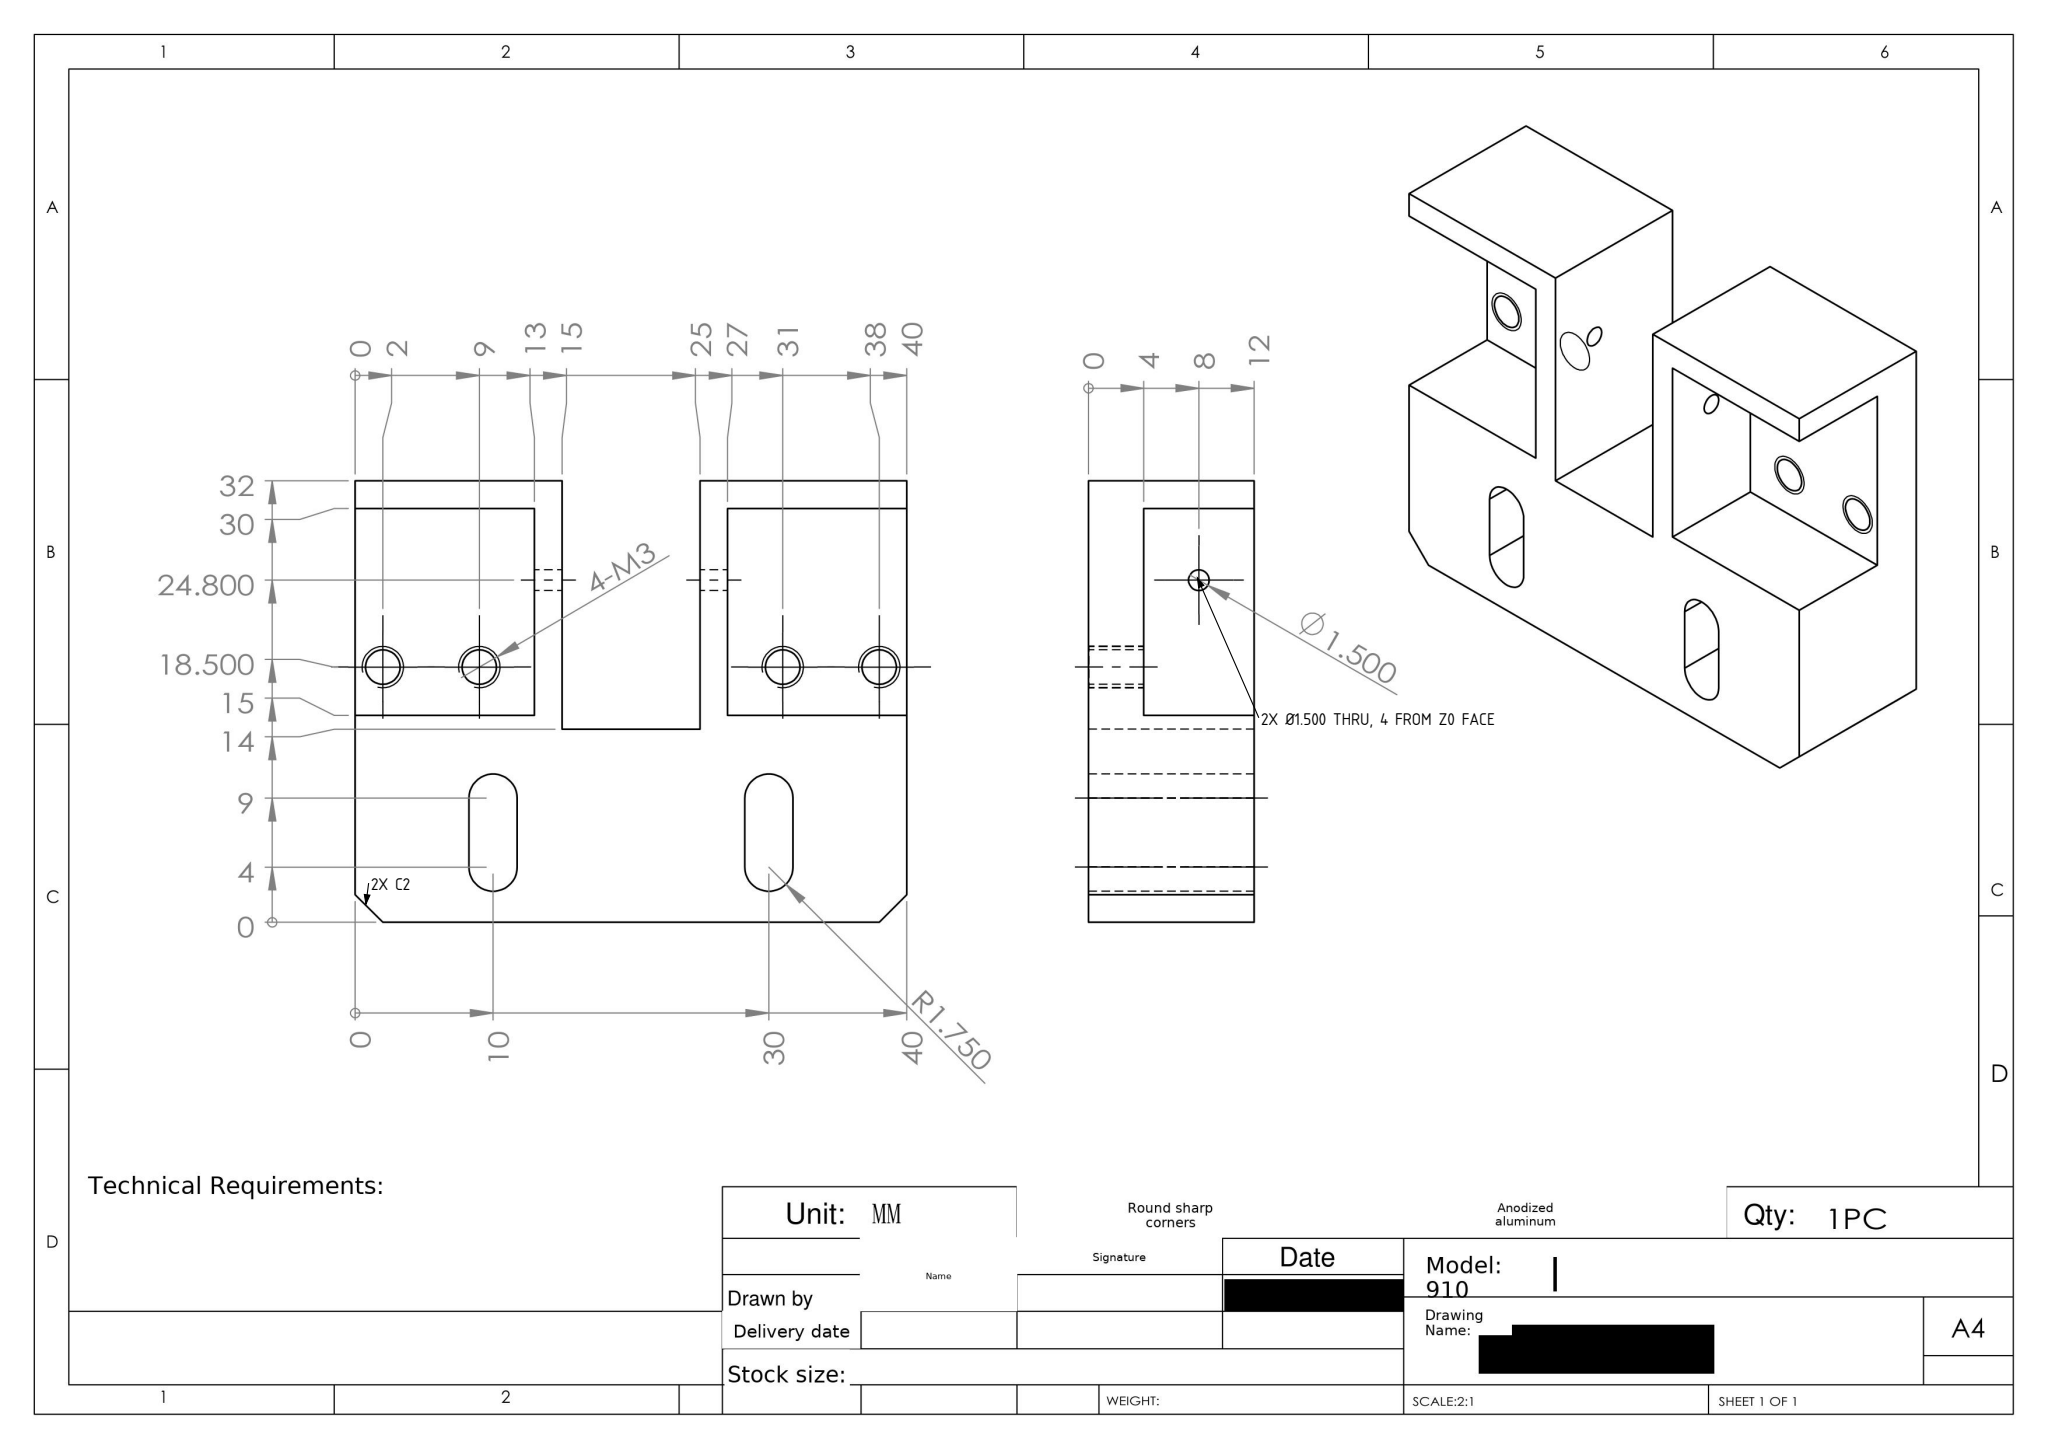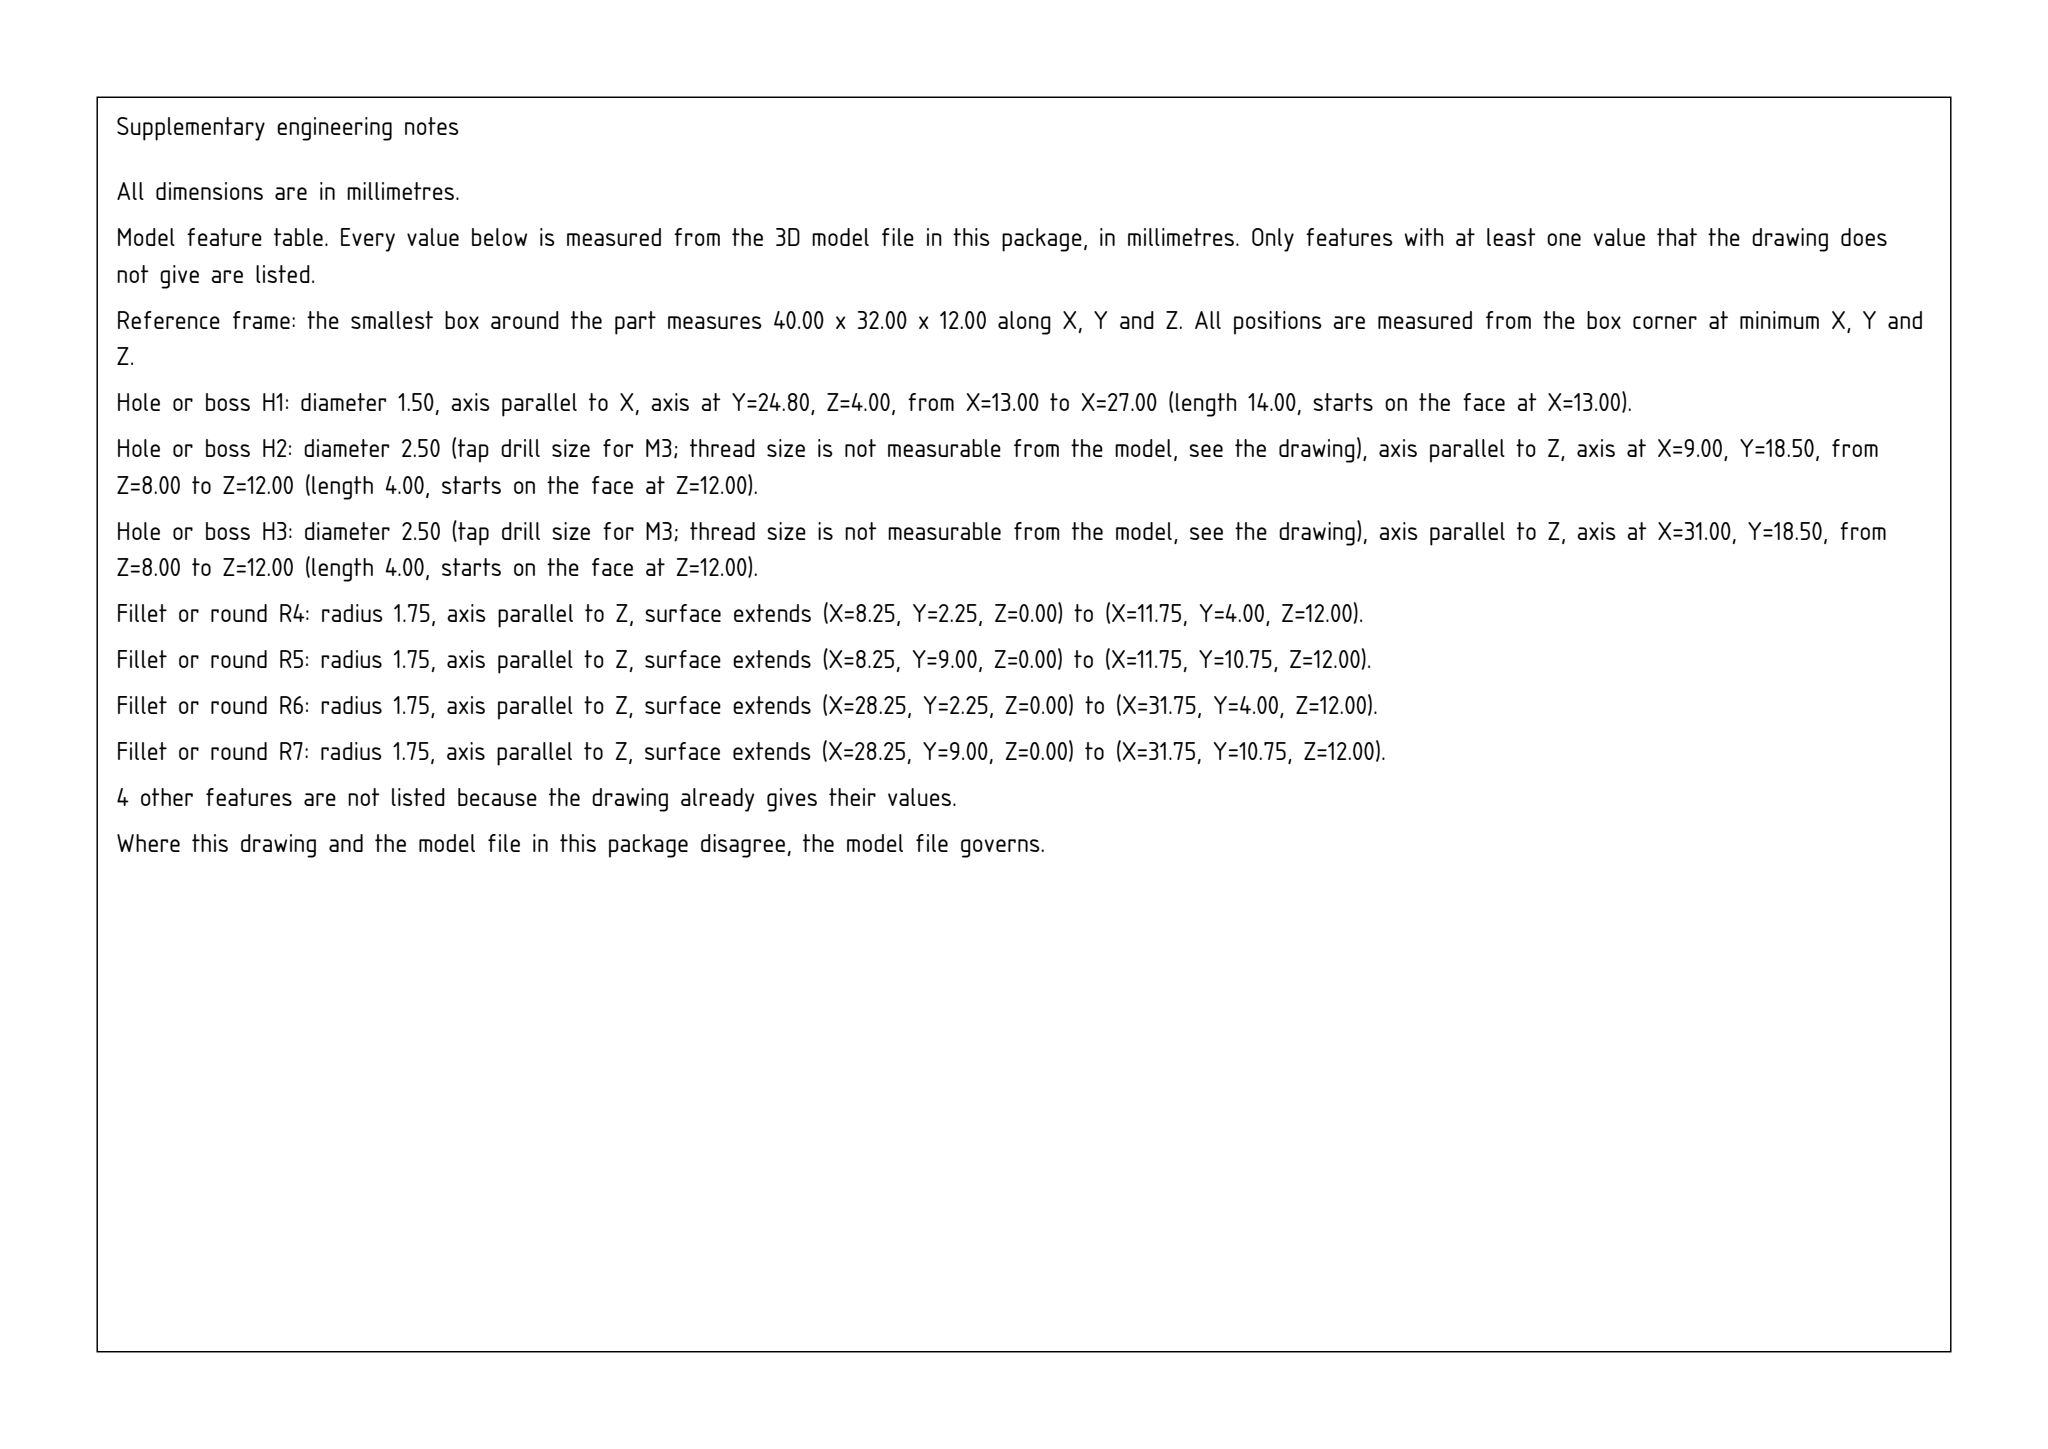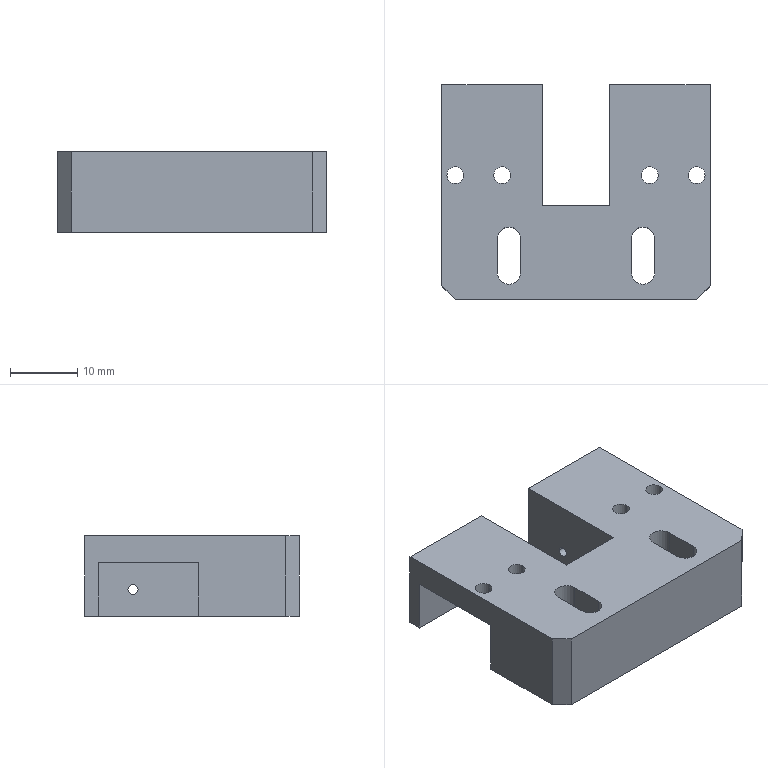Part | SolidWorks | mm | material Anodized aluminum | 1 solid | 40 faces | box 40 x 32 x 12 mm | volume 9295 mm3 | plane 24 | cylinder 16 | commonest cylinder face diameters 2.5 x8 1.5 x4 3.5 x4
Drawing notes:
2X Ø1.500 THRU 2 WALL, @ 24.800 FROM BTM, 4 FROM Z0 FACE | from the solid: cylinders dia 1.5 axis x at [y24.8,z4.0], x13-15 and x25-27 only (2 total)
2X C2 CHAMFER AT BOTTOM CORNERS (X0/Y0 AND X38/Y0) | from the solid: inclined_planes 45°, bbox_from [0,0,0] and [38,0,0], size 2.0 x 2.0 x 12.0